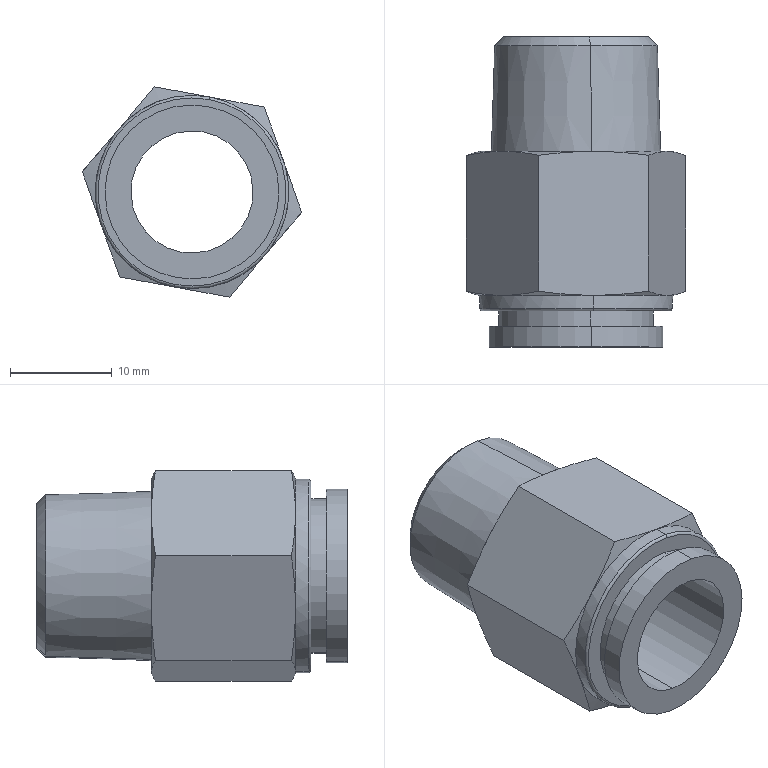Component | SolidWorks | A4-MLCNLSS12-3-L-1 | 1 solid | 37 faces | volume 4476 mm3 | cone 16 | plane 11 | cylinder 8 | torus 2 | commonest cylinder face diameters 12 x2 17.1 x2 15.2 x2 19 x2